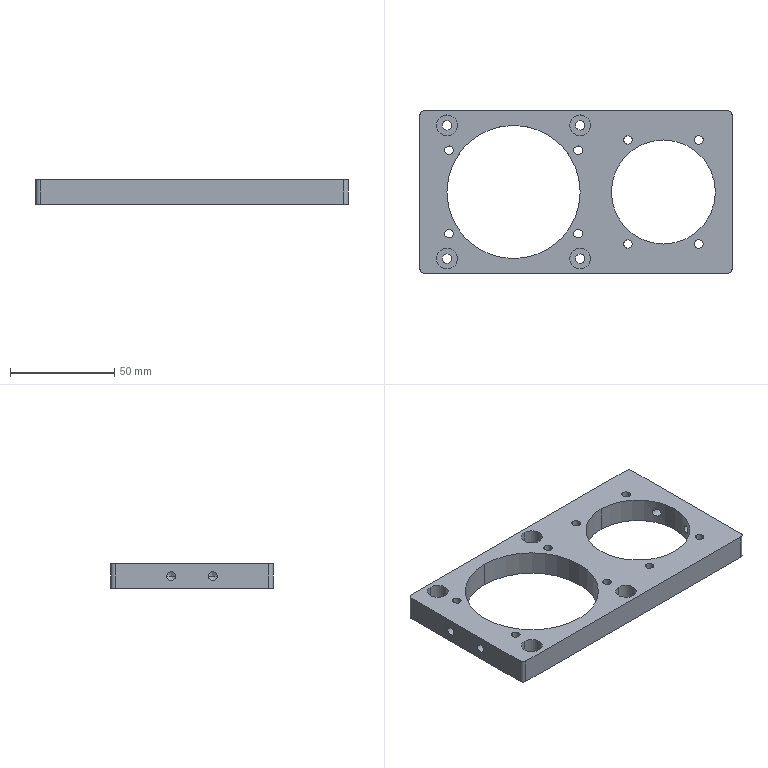CAM job | Mastercam | mm | 15 operations | part box 150 x 78 x 12
1. Facing | 20 - 63 平铣刀
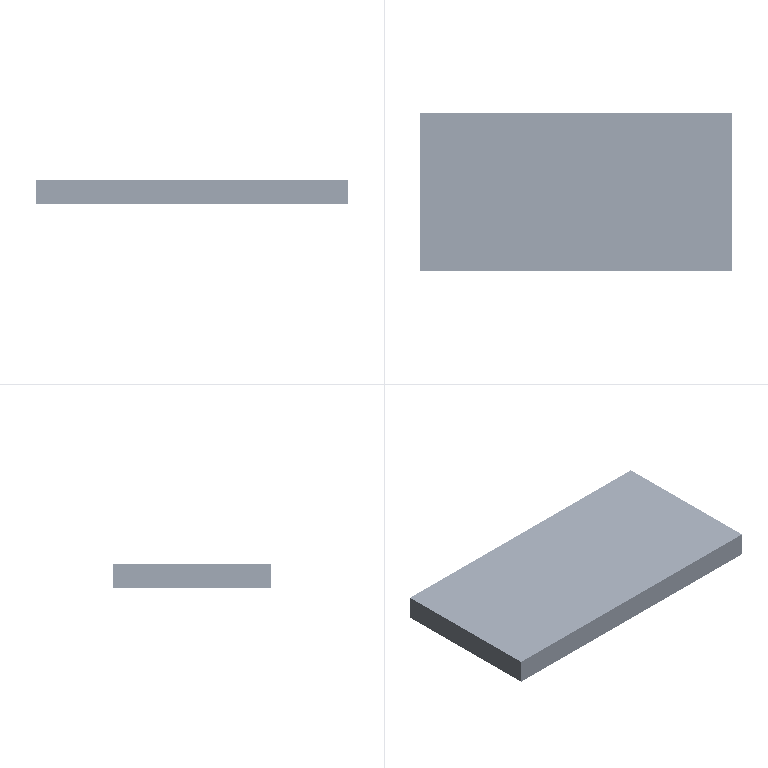2. Contour (Ramp) | 12 - 12 平铣刀
3. Contour (Ramp) | 12 - 12 平铣刀
4. Contour (2D) | 12 - 12 平铣刀
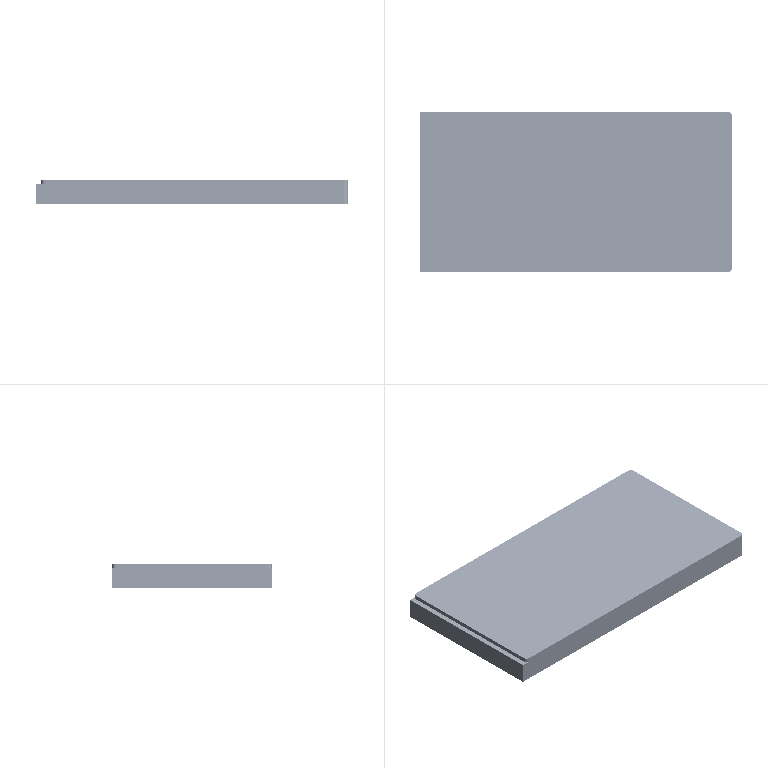5. 2D High Speed (2D Dynamic Mill) | 12 - 12 平铣刀
6. Contour (2D) | 12 - 12 平铣刀
7. Contour (Ramp) | 6 - 6 平铣刀
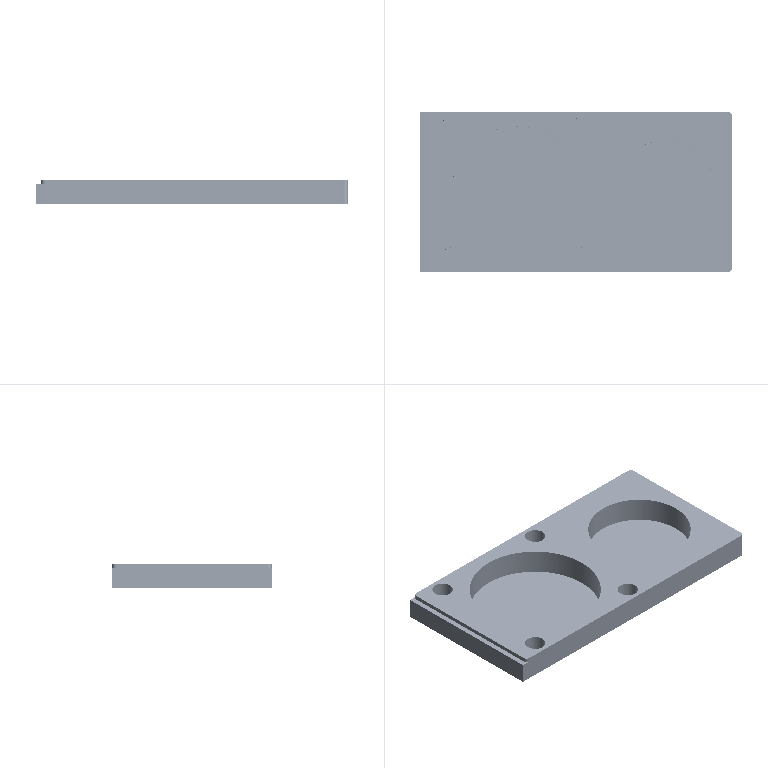8. Contour (Ramp) | 6 - 6 平铣刀
9. Drill/Counterbore | 7 - 4 倒角刀
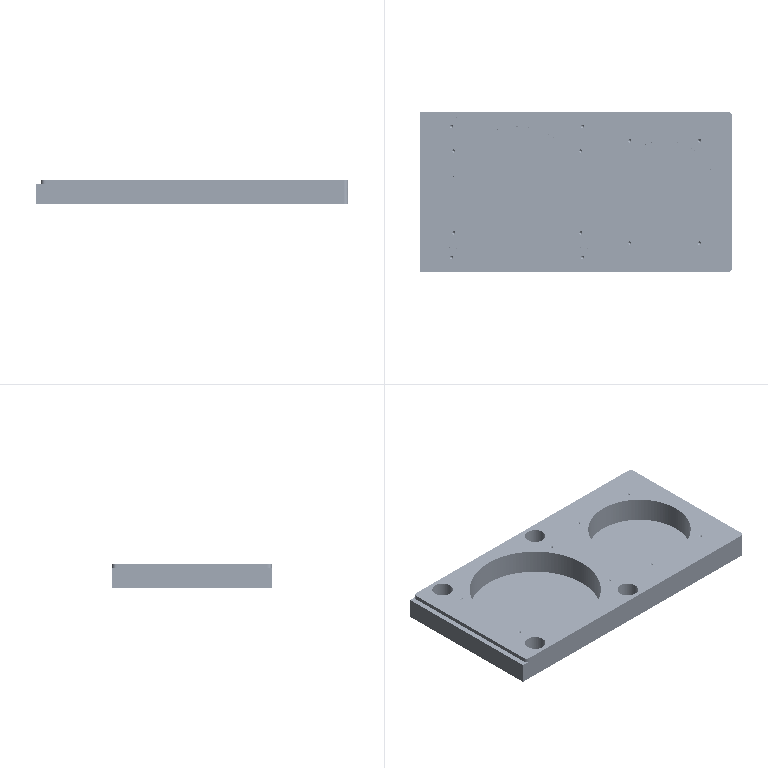10. Contour (2D chamfer) | 7 - 4 倒角刀
11. Contour (Ramp) | 12 - 12 平铣刀
12. Contour (2D) | 12 - 12 平铣刀
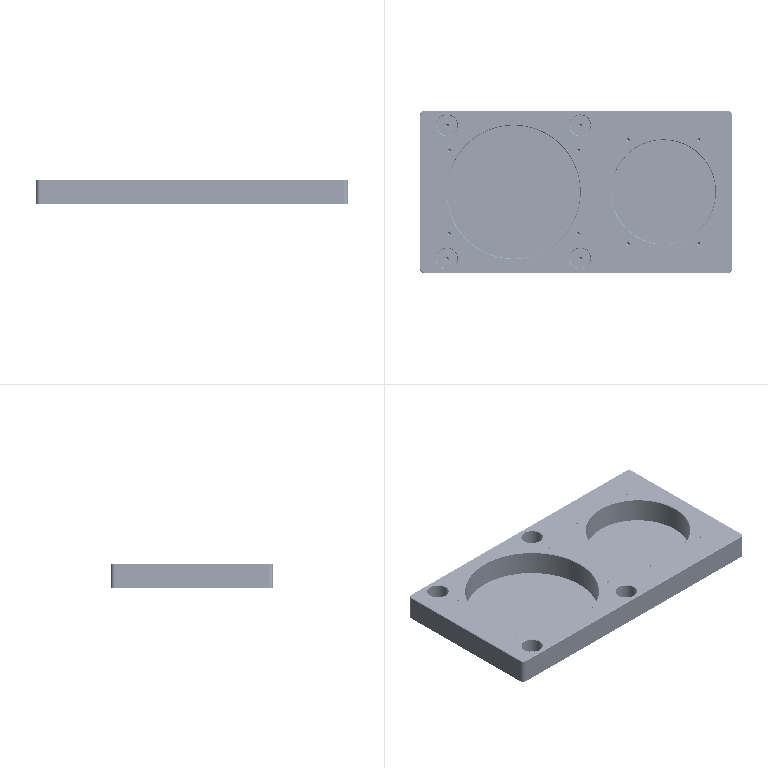13. Contour (2D chamfer) | 7 - 4 倒角刀
14. Drill/Counterbore | 7 - 4 倒角刀
15. Drill/Counterbore | 7 - 4 倒角刀